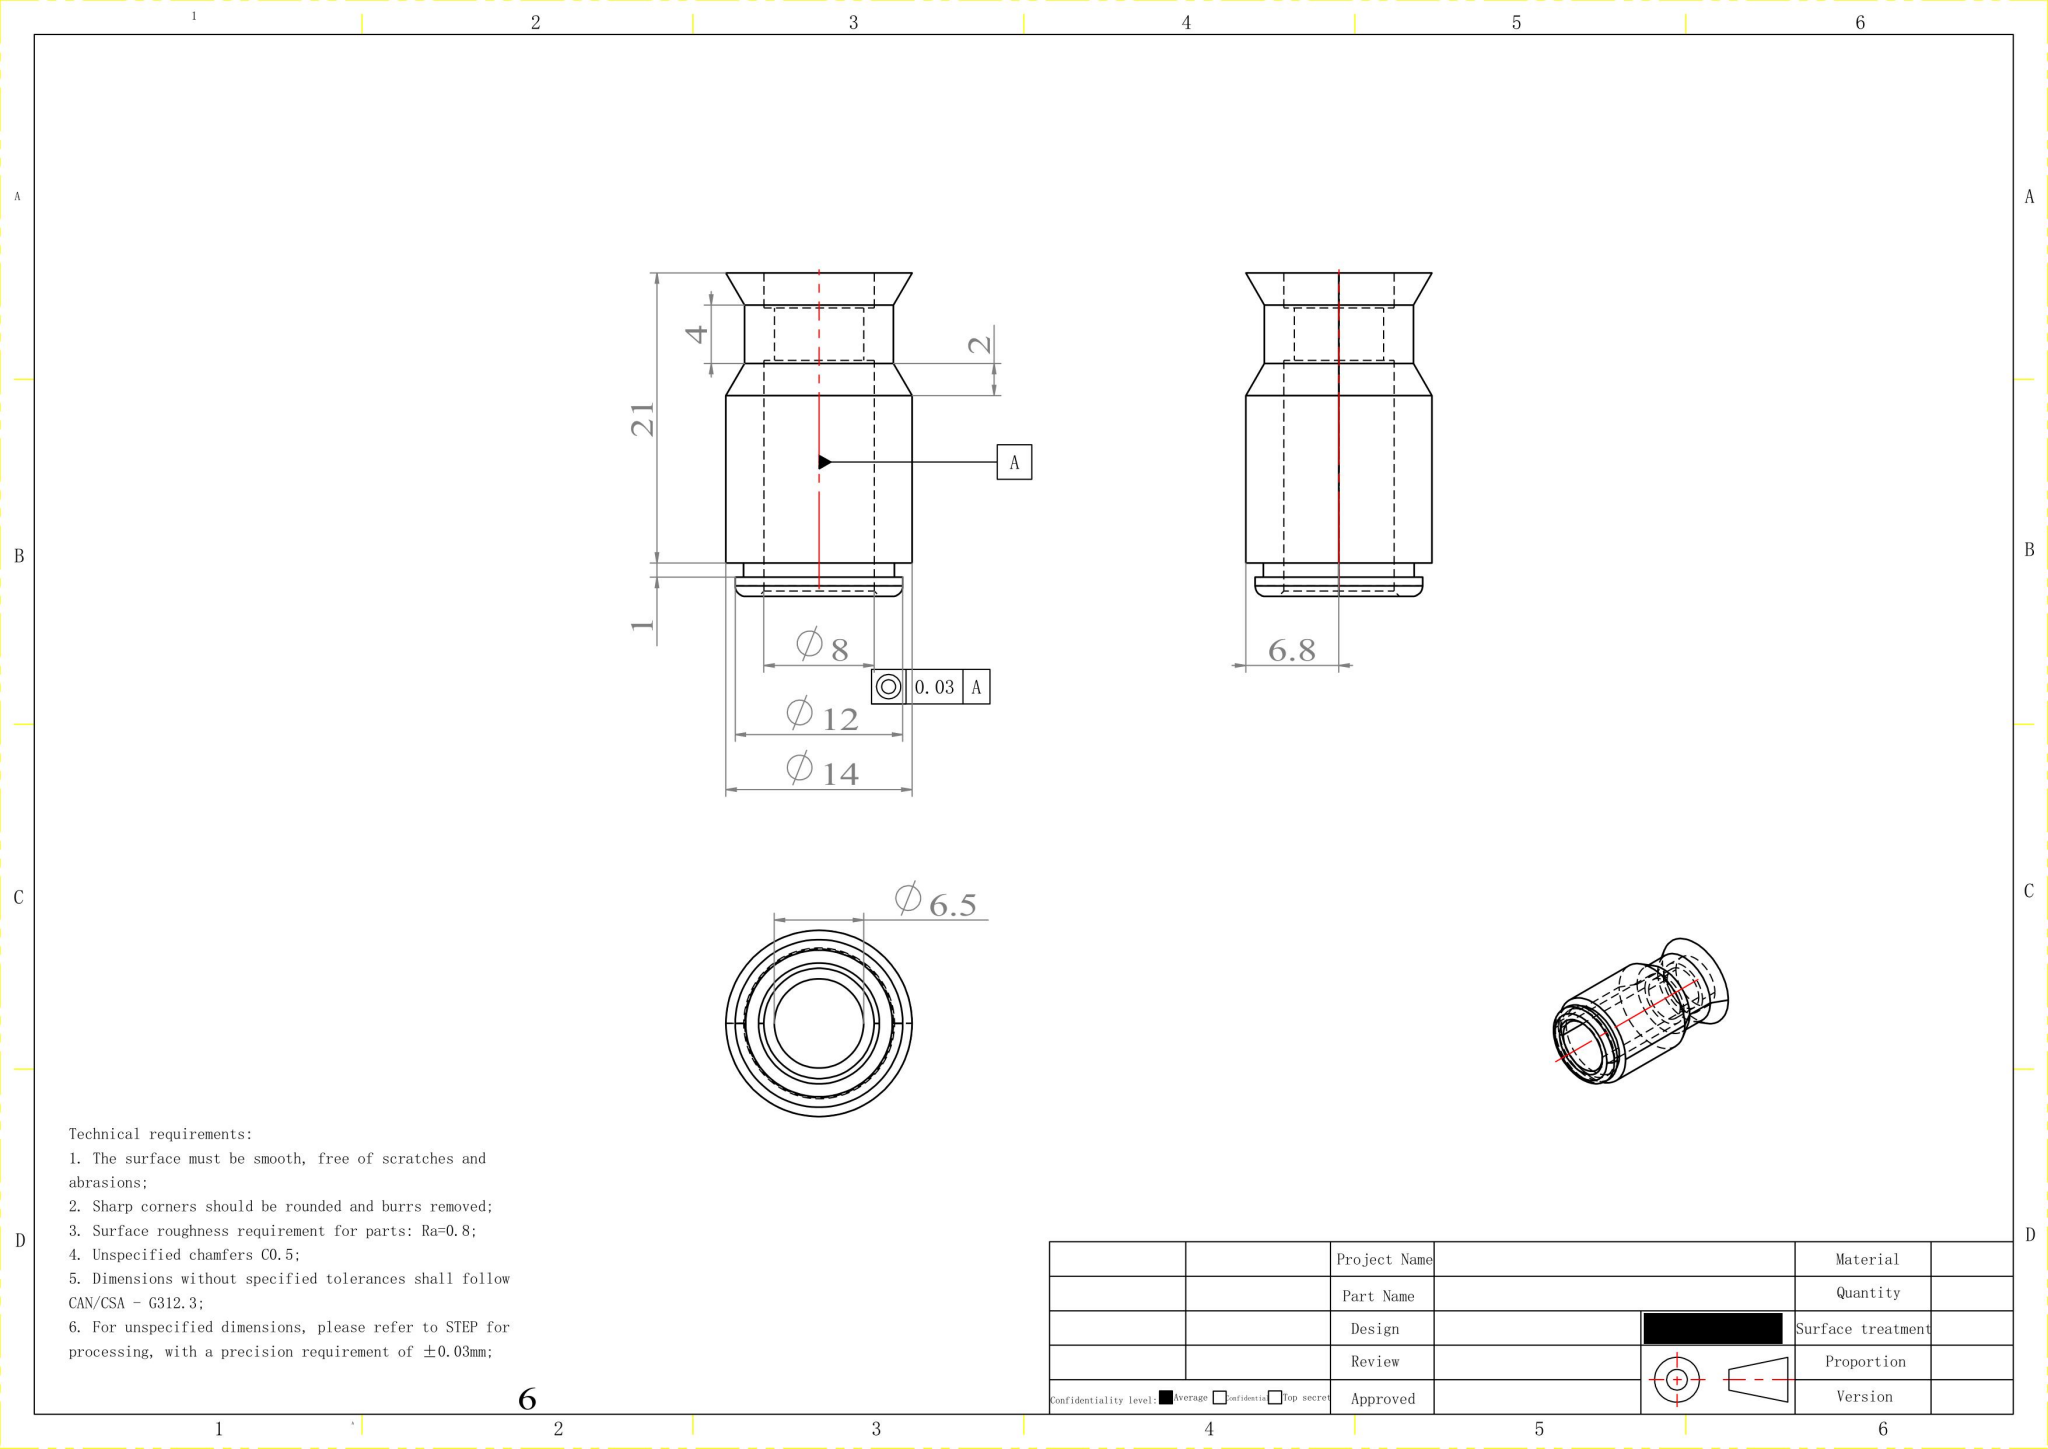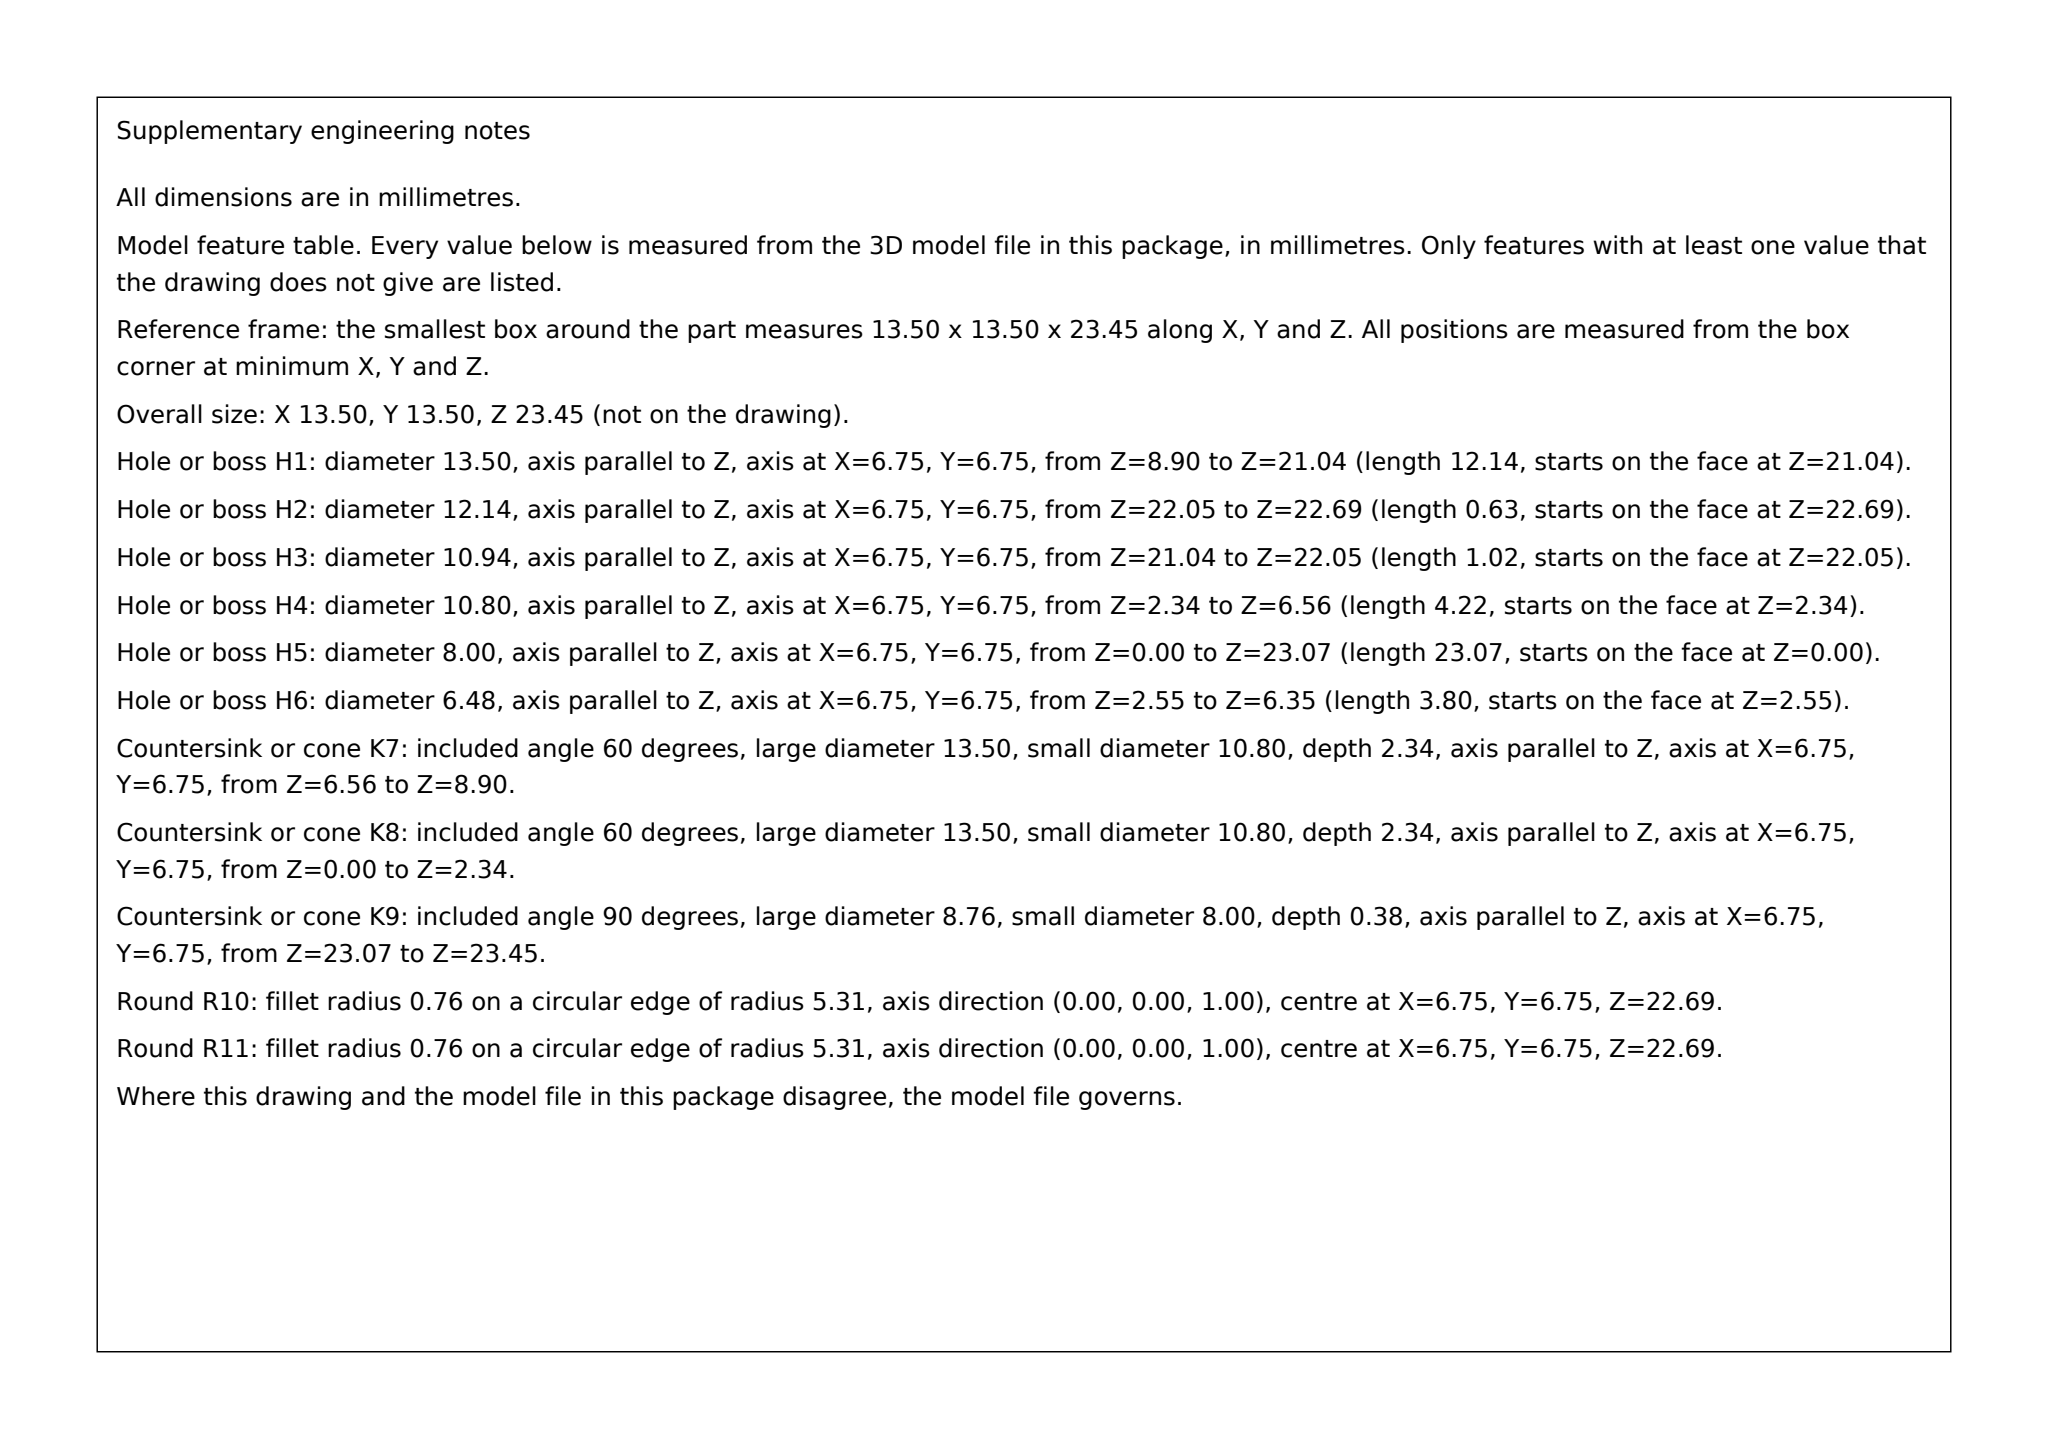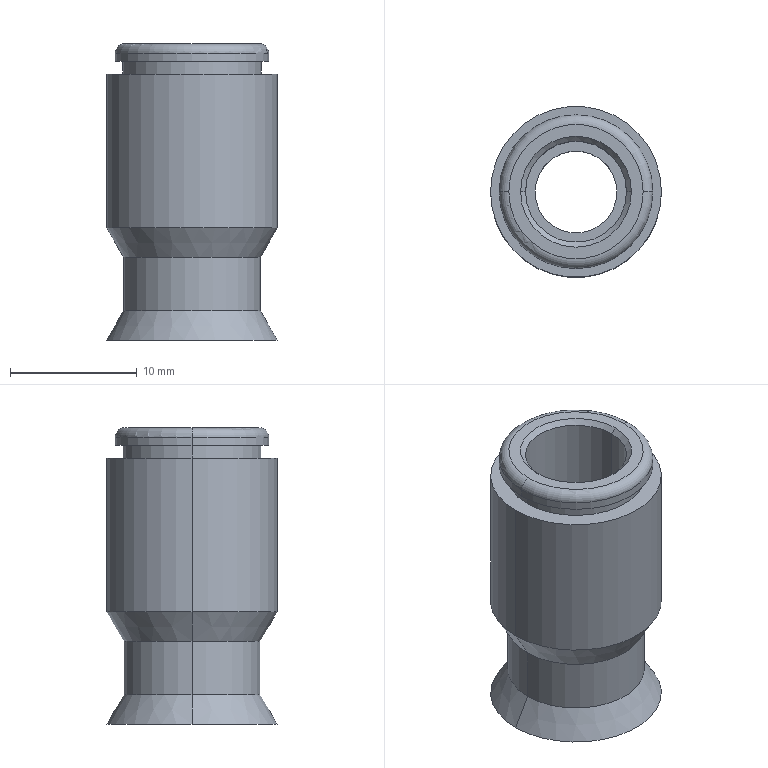Part | SolidWorks | mm | 1 solid | 28 faces | box 13.5 x 13.5 x 23.45 mm | volume 1807 mm3 | cylinder 14 | plane 6 | cone 6 | torus 2 | commonest cylinder face diameters 8 x4 6.476 x2 10.8 x2 13.5 x2 10.935 x2 12.15 x2
STEP:
#1=CARTESIAN_POINT('',(3.238,0.,1.9));
#2=VERTEX_POINT('',#1);
#3=CARTESIAN_POINT('',(-3.238,-0.,1.9));
#4=VERTEX_POINT('',#3);
#5=CARTESIAN_POINT('',(-0.,-0.,1.9));
#6=DIRECTION('',(0.,-0.,1.));
#7=DIRECTION('',(1.,0.,-0.));
#8=AXIS2_PLACEMENT_3D('',#5,#6,#7);
#9=CIRCLE('',#8,3.238);
#10=EDGE_CURVE('',#2,#4,#9,.T.);
#11=ORIENTED_EDGE('',*,*,#10,.F.);
#12=CARTESIAN_POINT('',(0.,0.,1.9));
#13=DIRECTION('',(-0.,0.,1.));
#14=DIRECTION('',(-1.,-0.,-0.));
#15=AXIS2_PLACEMENT_3D('',#12,#13,#14);
#16=CIRCLE('',#15,3.238);
#17=EDGE_CURVE('',#4,#2,#16,.T.);
#18=ORIENTED_EDGE('',*,*,#17,.F.);
#19=EDGE_LOOP('',(#11,#18));
#20=FACE_BOUND('',#19,.T.);
#21=CARTESIAN_POINT('',(4.,-0.,1.9));
#22=VERTEX_POINT('',#21);
#23=CARTESIAN_POINT('',(-4.,0.,1.9));
#24=VERTEX_POINT('',#23);
#25=CARTESIAN_POINT('',(0.,0.,1.9));
#26=DIRECTION('',(-0.,-0.,-1.));
#27=DIRECTION('',(1.,-0.,-0.));
#28=AXIS2_PLACEMENT_3D('',#25,#26,#27);
#29=CIRCLE('',#28,4.);
#30=EDGE_CURVE('',#22,#24,#29,.T.);
#31=ORIENTED_EDGE('',*,*,#30,.F.);
#32=CARTESIAN_POINT('',(0.,0.,1.9));
#33=DIRECTION('',(0.,0.,-1.));
#34=DIRECTION('',(-1.,0.,-0.));
#35=AXIS2_PLACEMENT_3D('',#32,#33,#34);
#36=CIRCLE('',#35,4.);
#37=EDGE_CURVE('',#24,#22,#36,.T.);
#38=ORIENTED_EDGE('',*,*,#37,.F.);
#39=EDGE_LOOP('',(#31,#38));
#40=FACE_OUTER_BOUND('',#39,.T.);
#41=CARTESIAN_POINT('',(0.,4.,1.9));
#42=DIRECTION('',(0.,0.,1.));
#43=DIRECTION('',(1.,0.,0.));
#44=AXIS2_PLACEMENT_3D('',#41,#42,#43);
#45=PLANE('',#44);
#46=ADVANCED_FACE('',(#20,#40),#45,.T.);
#47=CARTESIAN_POINT('',(-4.381,-0.,19.));
#48=VERTEX_POINT('',#47);
#49=CARTESIAN_POINT('',(4.381,0.,19.));
#50=VERTEX_POINT('',#49);
#51=CARTESIAN_POINT('',(0.,0.,19.));
#52=DIRECTION('',(0.,-0.,1.));
#53=DIRECTION('',(-1.,-0.,0.));
#54=AXIS2_PLACEMENT_3D('',#51,#52,#53);
#55=CIRCLE('',#54,4.381);
#56=EDGE_CURVE('',#48,#50,#55,.T.);
#57=ORIENTED_EDGE('',*,*,#56,.F.);
#58=CARTESIAN_POINT('',(0.,0.,19.));
#59=DIRECTION('',(0.,0.,1.));
#60=DIRECTION('',(1.,-0.,0.));
#61=AXIS2_PLACEMENT_3D('',#58,#59,#60);
#62=CIRCLE('',#61,4.381);
#63=EDGE_CURVE('',#50,#48,#62,.T.);
#64=ORIENTED_EDGE('',*,*,#63,.F.);
#65=EDGE_LOOP('',(#57,#64));
#66=FACE_BOUND('',#65,.T.);
#67=CARTESIAN_POINT('',(5.313,0.,19.));
#68=VERTEX_POINT('',#67);
#69=CARTESIAN_POINT('',(-5.313,0.,19.));
#70=VERTEX_POINT('',#69);
#71=CARTESIAN_POINT('',(0.,-0.,19.));
#72=DIRECTION('',(-0.,-0.,-1.));
#73=DIRECTION('',(1.,0.,-0.));
#74=AXIS2_PLACEMENT_3D('',#71,#72,#73);
#75=CIRCLE('',#74,5.313);
#76=EDGE_CURVE('',#68,#70,#75,.T.);
#77=ORIENTED_EDGE('',*,*,#76,.F.);
#78=CARTESIAN_POINT('',(0.,-0.,19.));
#79=DIRECTION('',(-0.,-0.,-1.));
#80=DIRECTION('',(-1.,0.,0.));
#81=AXIS2_PLACEMENT_3D('',#78,#79,#80);
#82=CIRCLE('',#81,5.313);
#83=EDGE_CURVE('',#70,#68,#82,.T.);
#84=ORIENTED_EDGE('',*,*,#83,.F.);
#85=EDGE_LOOP('',(#77,#84));
#86=FACE_OUTER_BOUND('',#85,.T.);
#87=CARTESIAN_POINT('',(0.,5.313,19.));
#88=DIRECTION('',(0.,0.,1.));
#89=DIRECTION('',(1.,0.,0.));
#90=AXIS2_PLACEMENT_3D('',#87,#88,#89);
#91=PLANE('',#90);
#92=ADVANCED_FACE('',(#66,#86),#91,.T.);
#93=CARTESIAN_POINT('',(5.468,0.,17.603));
#94=VERTEX_POINT('',#93);
#95=CARTESIAN_POINT('',(-5.468,0.,17.603));
#96=VERTEX_POINT('',#95);
#97=CARTESIAN_POINT('',(0.,-0.,17.603));
#98=DIRECTION('',(0.,0.,-1.));
#99=DIRECTION('',(1.,-0.,0.));
#100=AXIS2_PLACEMENT_3D('',#97,#98,#99);
#101=CIRCLE('',#100,5.468);
#102=EDGE_CURVE('',#94,#96,#101,.T.);
#103=ORIENTED_EDGE('',*,*,#102,.F.);
#104=CARTESIAN_POINT('',(0.,-0.,17.603));
#105=DIRECTION('',(-0.,-0.,-1.));
#106=DIRECTION('',(-1.,0.,0.));
#107=AXIS2_PLACEMENT_3D('',#104,#105,#106);
#108=CIRCLE('',#107,5.468);
#109=EDGE_CURVE('',#96,#94,#108,.T.);
#110=ORIENTED_EDGE('',*,*,#109,.F.);
#111=EDGE_LOOP('',(#103,#110));
#112=FACE_BOUND('',#111,.T.);
#113=CARTESIAN_POINT('',(6.075,-0.,17.603));
#114=VERTEX_POINT('',#113);
#115=CARTESIAN_POINT('',(-6.075,0.,17.603));
#116=VERTEX_POINT('',#115);
#117=CARTESIAN_POINT('',(0.,0.,17.603));
#118=DIRECTION('',(-0.,-0.,1.));
#119=DIRECTION('',(1.,-0.,0.));
#120=AXIS2_PLACEMENT_3D('',#117,#118,#119);
#121=CIRCLE('',#120,6.075);
#122=EDGE_CURVE('',#114,#116,#121,.T.);
#123=ORIENTED_EDGE('',*,*,#122,.F.);
#124=CARTESIAN_POINT('',(0.,0.,17.603));
#125=DIRECTION('',(-0.,-0.,1.));
#126=DIRECTION('',(-1.,0.,0.));
#127=AXIS2_PLACEMENT_3D('',#124,#125,#126);
#128=CIRCLE('',#127,6.075);
#129=EDGE_CURVE('',#116,#114,#128,.T.);
#130=ORIENTED_EDGE('',*,*,#129,.F.);
#131=EDGE_LOOP('',(#123,#130));
#132=FACE_OUTER_BOUND('',#131,.T.);
#133=CARTESIAN_POINT('',(0.,6.075,17.603));
#134=DIRECTION('',(0.,0.,-1.));
#135=DIRECTION('',(0.,-1.,0.));
#136=AXIS2_PLACEMENT_3D('',#133,#134,#135);
#137=PLANE('',#136);
#138=ADVANCED_FACE('',(#112,#132),#137,.T.);
#139=CARTESIAN_POINT('',(5.468,-0.,16.587));
#140=VERTEX_POINT('',#139);
#141=CARTESIAN_POINT('',(-5.468,0.,16.587));
#142=VERTEX_POINT('',#141);
#143=CARTESIAN_POINT('',(0.,-0.,16.587));
#144=DIRECTION('',(0.,0.,1.));
#145=DIRECTION('',(1.,-0.,0.));
#146=AXIS2_PLACEMENT_3D('',#143,#144,#145);
#147=CIRCLE('',#146,5.468);
#148=EDGE_CURVE('',#140,#142,#147,.T.);
#149=ORIENTED_EDGE('',*,*,#148,.F.);
#150=CARTESIAN_POINT('',(-0.,-0.,16.587));
#151=DIRECTION('',(0.,0.,1.));
#152=DIRECTION('',(-1.,0.,0.));
#153=AXIS2_PLACEMENT_3D('',#150,#151,#152);
#154=CIRCLE('',#153,5.468);
#155=EDGE_CURVE('',#142,#140,#154,.T.);
#156=ORIENTED_EDGE('',*,*,#155,.F.);
#157=EDGE_LOOP('',(#149,#156));
#158=FACE_BOUND('',#157,.T.);
#159=CARTESIAN_POINT('',(6.75,0.,16.587));
#160=VERTEX_POINT('',#159);
#161=CARTESIAN_POINT('',(-6.75,0.,16.587));
#162=VERTEX_POINT('',#161);
#163=CARTESIAN_POINT('',(0.,0.,16.587));
#164=DIRECTION('',(0.,0.,-1.));
#165=DIRECTION('',(1.,-0.,0.));
#166=AXIS2_PLACEMENT_3D('',#163,#164,#165);
#167=CIRCLE('',#166,6.75);
#168=EDGE_CURVE('',#160,#162,#167,.T.);
#169=ORIENTED_EDGE('',*,*,#168,.F.);
#170=CARTESIAN_POINT('',(0.,0.,16.587));
#171=DIRECTION('',(0.,0.,-1.));
#172=DIRECTION('',(-1.,0.,0.));
#173=AXIS2_PLACEMENT_3D('',#170,#171,#172);
#174=CIRCLE('',#173,6.75);
#175=EDGE_CURVE('',#162,#160,#174,.T.);
#176=ORIENTED_EDGE('',*,*,#175,.F.);
#177=EDGE_LOOP('',(#169,#176));
#178=FACE_OUTER_BOUND('',#177,.T.);
#179=CARTESIAN_POINT('',(0.,6.75,16.587));
#180=DIRECTION('',(0.,0.,1.));
#181=DIRECTION('',(1.,0.,0.));
#182=AXIS2_PLACEMENT_3D('',#179,#180,#181);
#183=PLANE('',#182);
#184=ADVANCED_FACE('',(#158,#178),#183,.T.);
#185=CARTESIAN_POINT('',(3.238,0.,-1.9));
#186=VERTEX_POINT('',#185);
#187=CARTESIAN_POINT('',(-3.238,-0.,-1.9));
#188=VERTEX_POINT('',#187);
#189=CARTESIAN_POINT('',(-0.,-0.,-1.9));
#190=DIRECTION('',(0.,-0.,-1.));
#191=DIRECTION('',(1.,0.,0.));
#192=AXIS2_PLACEMENT_3D('',#189,#190,#191);
#193=CIRCLE('',#192,3.238);
#194=EDGE_CURVE('',#186,#188,#193,.T.);
#195=ORIENTED_EDGE('',*,*,#194,.F.);
#196=CARTESIAN_POINT('',(0.,0.,-1.9));
#197=DIRECTION('',(-0.,-0.,-1.));
#198=DIRECTION('',(-1.,-0.,0.));
#199=AXIS2_PLACEMENT_3D('',#196,#197,#198);
#200=CIRCLE('',#199,3.238);
#201=EDGE_CURVE('',#188,#186,#200,.T.);
#202=ORIENTED_EDGE('',*,*,#201,.F.);
#203=EDGE_LOOP('',(#195,#202));
#204=FACE_BOUND('',#203,.T.);
#205=CARTESIAN_POINT('',(4.,-0.,-1.9));
#206=VERTEX_POINT('',#205);
#207=CARTESIAN_POINT('',(-4.,-0.,-1.9));
#208=VERTEX_POINT('',#207);
#209=CARTESIAN_POINT('',(0.,-0.,-1.9));
#210=DIRECTION('',(-0.,-0.,1.));
#211=DIRECTION('',(1.,0.,0.));
#212=AXIS2_PLACEMENT_3D('',#209,#210,#211);
#213=CIRCLE('',#212,4.);
#214=EDGE_CURVE('',#206,#208,#213,.T.);
#215=ORIENTED_EDGE('',*,*,#214,.F.);
#216=CARTESIAN_POINT('',(-0.,-0.,-1.9));
#217=DIRECTION('',(0.,-0.,1.));
#218=DIRECTION('',(-1.,0.,0.));
#219=AXIS2_PLACEMENT_3D('',#216,#217,#218);
#220=CIRCLE('',#219,4.);
#221=EDGE_CURVE('',#208,#206,#220,.T.);
#222=ORIENTED_EDGE('',*,*,#221,.F.);
#223=EDGE_LOOP('',(#215,#222));
#224=FACE_OUTER_BOUND('',#223,.T.);
#225=CARTESIAN_POINT('',(0.,4.,-1.9));
#226=DIRECTION('',(0.,0.,-1.));
#227=DIRECTION('',(0.,-1.,0.));
#228=AXIS2_PLACEMENT_3D('',#225,#226,#227);
#229=PLANE('',#228);
#230=ADVANCED_FACE('',(#204,#224),#229,.T.);
#231=CARTESIAN_POINT('',(-6.75,-0.,-4.449));
#232=VERTEX_POINT('',#231);
#233=CARTESIAN_POINT('',(6.75,0.,-4.449));
#234=VERTEX_POINT('',#233);
#235=CARTESIAN_POINT('',(0.,0.,-4.449));
#236=DIRECTION('',(0.,0.,-1.));
#237=DIRECTION('',(-1.,-0.,0.));
#238=AXIS2_PLACEMENT_3D('',#235,#236,#237);
#239=CIRCLE('',#238,6.75);
#240=EDGE_CURVE('',#232,#234,#239,.T.);
#241=ORIENTED_EDGE('',*,*,#240,.F.);
#242=CARTESIAN_POINT('',(-5.4,-0.,-2.111));
#243=VERTEX_POINT('',#242);
#244=CARTESIAN_POINT('',(-5.4,0.,-2.111));
#245=DIRECTION('',(-0.5,0.,-0.866));
#246=VECTOR('',#245,1000.);
#247=LINE('',#244,#246);
#248=EDGE_CURVE('',#243,#232,#247,.T.);
#249=ORIENTED_EDGE('',*,*,#248,.F.);
#250=CARTESIAN_POINT('',(5.4,0.,-2.111));
#251=VERTEX_POINT('',#250);
#252=CARTESIAN_POINT('',(0.,0.,-2.111));
#253=DIRECTION('',(-0.,0.,1.));
#254=DIRECTION('',(1.,0.,0.));
#255=AXIS2_PLACEMENT_3D('',#252,#253,#254);
#256=CIRCLE('',#255,5.4);
#257=EDGE_CURVE('',#251,#243,#256,.T.);
#258=ORIENTED_EDGE('',*,*,#257,.F.);
#259=CARTESIAN_POINT('',(6.75,0.,-4.449));
#260=DIRECTION('',(-0.5,-0.,0.866));
#261=VECTOR('',#260,1000.);
#262=LINE('',#259,#261);
#263=EDGE_CURVE('',#234,#251,#262,.T.);
#264=ORIENTED_EDGE('',*,*,#263,.F.);
#265=EDGE_LOOP('',(#241,#249,#258,#264));
#266=FACE_OUTER_BOUND('',#265,.T.);
#267=CARTESIAN_POINT('',(0.,0.,6.242));
#268=DIRECTION('',(0.,0.,-1.));
#269=DIRECTION('',(-1.,-0.,0.));
#270=AXIS2_PLACEMENT_3D('',#267,#268,#269);
#271=CONICAL_SURFACE('',#270,0.5774,0.5236);
#272=ADVANCED_FACE('',(#266),#271,.T.);
#273=ORIENTED_EDGE('',*,*,#263,.T.);
#274=CARTESIAN_POINT('',(-0.,-0.,-2.111));
#275=DIRECTION('',(0.,-0.,1.));
#276=DIRECTION('',(-1.,-0.,0.));
#277=AXIS2_PLACEMENT_3D('',#274,#275,#276);
#278=CIRCLE('',#277,5.4);
#279=EDGE_CURVE('',#243,#251,#278,.T.);
#280=ORIENTED_EDGE('',*,*,#279,.F.);
#281=ORIENTED_EDGE('',*,*,#248,.T.);
#282=CARTESIAN_POINT('',(-0.,0.,-4.449));
#283=DIRECTION('',(0.,0.,-1.));
#284=DIRECTION('',(1.,-0.,0.));
#285=AXIS2_PLACEMENT_3D('',#282,#283,#284);
#286=CIRCLE('',#285,6.75);
#287=EDGE_CURVE('',#234,#232,#286,.T.);
#288=ORIENTED_EDGE('',*,*,#287,.F.);
#289=EDGE_LOOP('',(#273,#280,#281,#288));
#290=FACE_OUTER_BOUND('',#289,.T.);
#291=CARTESIAN_POINT('',(0.,0.,6.242));
#292=DIRECTION('',(0.,0.,-1.));
#293=DIRECTION('',(-1.,-0.,0.));
#294=AXIS2_PLACEMENT_3D('',#291,#292,#293);
#295=CONICAL_SURFACE('',#294,0.5774,0.5236);
#296=ADVANCED_FACE('',(#290),#295,.T.);
#297=CARTESIAN_POINT('',(4.,0.,-4.449));
#298=VERTEX_POINT('',#297);
#299=CARTESIAN_POINT('',(-4.,0.,-4.449));
#300=VERTEX_POINT('',#299);
#301=CARTESIAN_POINT('',(0.,-0.,-4.449));
#302=DIRECTION('',(0.,0.,1.));
#303=DIRECTION('',(1.,-0.,0.));
#304=AXIS2_PLACEMENT_3D('',#301,#302,#303);
#305=CIRCLE('',#304,4.);
#306=EDGE_CURVE('',#298,#300,#305,.T.);
#307=ORIENTED_EDGE('',*,*,#306,.F.);
#308=CARTESIAN_POINT('',(4.,0.,-1.9));
#309=DIRECTION('',(0.,0.,-1.));
#310=VECTOR('',#309,1000.);
#311=LINE('',#308,#310);
#312=EDGE_CURVE('',#206,#298,#311,.T.);
#313=ORIENTED_EDGE('',*,*,#312,.F.);
#314=ORIENTED_EDGE('',*,*,#214,.T.);
#315=CARTESIAN_POINT('',(-4.,0.,-4.449));
#316=DIRECTION('',(0.,-0.,1.));
#317=VECTOR('',#316,1000.);
#318=LINE('',#315,#317);
#319=EDGE_CURVE('',#300,#208,#318,.T.);
#320=ORIENTED_EDGE('',*,*,#319,.F.);
#321=EDGE_LOOP('',(#307,#313,#314,#320));
#322=FACE_OUTER_BOUND('',#321,.T.);
#323=CARTESIAN_POINT('',(0.,-0.,-4.449));
#324=DIRECTION('',(-0.,0.,1.));
#325=DIRECTION('',(1.,0.,0.));
#326=AXIS2_PLACEMENT_3D('',#323,#324,#325);
#327=CYLINDRICAL_SURFACE('',#326,4.);
#328=ADVANCED_FACE('',(#322),#327,.F.);
#329=ORIENTED_EDGE('',*,*,#319,.T.);
#330=ORIENTED_EDGE('',*,*,#221,.T.);
#331=ORIENTED_EDGE('',*,*,#312,.T.);
#332=CARTESIAN_POINT('',(-0.,-0.,-4.449));
#333=DIRECTION('',(0.,0.,1.));
#334=DIRECTION('',(-1.,0.,0.));
#335=AXIS2_PLACEMENT_3D('',#332,#333,#334);
#336=CIRCLE('',#335,4.);
#337=EDGE_CURVE('',#300,#298,#336,.T.);
#338=ORIENTED_EDGE('',*,*,#337,.F.);
#339=EDGE_LOOP('',(#329,#330,#331,#338));
#340=FACE_OUTER_BOUND('',#339,.T.);
#341=CARTESIAN_POINT('',(0.,-0.,-4.449));
#342=DIRECTION('',(-0.,0.,1.));
#343=DIRECTION('',(1.,0.,0.));
#344=AXIS2_PLACEMENT_3D('',#341,#342,#343);
#345=CYLINDRICAL_SURFACE('',#344,4.);
#346=ADVANCED_FACE('',(#340),#345,.F.);
#347=ORIENTED_EDGE('',*,*,#201,.T.);
#348=CARTESIAN_POINT('',(3.238,0.,1.9));
#349=DIRECTION('',(0.,0.,-1.));
#350=VECTOR('',#349,1000.);
#351=LINE('',#348,#350);
#352=EDGE_CURVE('',#2,#186,#351,.T.);
#353=ORIENTED_EDGE('',*,*,#352,.F.);
#354=ORIENTED_EDGE('',*,*,#10,.T.);
#355=CARTESIAN_POINT('',(-3.238,-0.,-1.9));
#356=DIRECTION('',(0.,0.,1.));
#357=VECTOR('',#356,1000.);
#358=LINE('',#355,#357);
#359=EDGE_CURVE('',#188,#4,#358,.T.);
#360=ORIENTED_EDGE('',*,*,#359,.F.);
#361=EDGE_LOOP('',(#347,#353,#354,#360));
#362=FACE_OUTER_BOUND('',#361,.T.);
#363=CARTESIAN_POINT('',(0.,0.,-1.9));
#364=DIRECTION('',(-0.,0.,1.));
#365=DIRECTION('',(1.,-0.,0.));
#366=AXIS2_PLACEMENT_3D('',#363,#364,#365);
#367=CYLINDRICAL_SURFACE('',#366,3.238);
#368=ADVANCED_FACE('',(#362),#367,.F.);
#369=ORIENTED_EDGE('',*,*,#359,.T.);
#370=ORIENTED_EDGE('',*,*,#17,.T.);
#371=ORIENTED_EDGE('',*,*,#352,.T.);
#372=ORIENTED_EDGE('',*,*,#194,.T.);
#373=EDGE_LOOP('',(#369,#370,#371,#372));
#374=FACE_OUTER_BOUND('',#373,.T.);
#375=CARTESIAN_POINT('',(0.,0.,-1.9));
#376=DIRECTION('',(-0.,0.,1.));
#377=DIRECTION('',(1.,-0.,0.));
#378=AXIS2_PLACEMENT_3D('',#375,#376,#377);
#379=CYLINDRICAL_SURFACE('',#378,3.238);
#380=ADVANCED_FACE('',(#374),#379,.F.);
#381=CARTESIAN_POINT('',(-5.4,0.,2.111));
#382=VERTEX_POINT('',#381);
#383=CARTESIAN_POINT('',(5.4,0.,2.111));
#384=VERTEX_POINT('',#383);
#385=CARTESIAN_POINT('',(-0.,-0.,2.111));
#386=DIRECTION('',(0.,0.,1.));
#387=DIRECTION('',(-1.,0.,0.));
#388=AXIS2_PLACEMENT_3D('',#385,#386,#387);
#389=CIRCLE('',#388,5.4);
#390=EDGE_CURVE('',#382,#384,#389,.T.);
#391=ORIENTED_EDGE('',*,*,#390,.F.);
#392=CARTESIAN_POINT('',(-5.4,0.,2.111));
#393=DIRECTION('',(0.,-0.,-1.));
#394=VECTOR('',#393,1000.);
#395=LINE('',#392,#394);
#396=EDGE_CURVE('',#382,#243,#395,.T.);
#397=ORIENTED_EDGE('',*,*,#396,.T.);
#398=ORIENTED_EDGE('',*,*,#279,.T.);
#399=CARTESIAN_POINT('',(5.4,0.,2.111));
#400=DIRECTION('',(0.,0.,-1.));
#401=VECTOR('',#400,1000.);
#402=LINE('',#399,#401);
#403=EDGE_CURVE('',#384,#251,#402,.T.);
#404=ORIENTED_EDGE('',*,*,#403,.F.);
#405=EDGE_LOOP('',(#391,#397,#398,#404));
#406=FACE_OUTER_BOUND('',#405,.T.);
#407=CARTESIAN_POINT('',(0.,-0.,-2.111));
#408=DIRECTION('',(-0.,-0.,1.));
#409=DIRECTION('',(1.,0.,0.));
#410=AXIS2_PLACEMENT_3D('',#407,#408,#409);
#411=CYLINDRICAL_SURFACE('',#410,5.4);
#412=ADVANCED_FACE('',(#406),#411,.T.);
#413=ORIENTED_EDGE('',*,*,#257,.T.);
#414=ORIENTED_EDGE('',*,*,#396,.F.);
#415=CARTESIAN_POINT('',(0.,0.,2.111));
#416=DIRECTION('',(0.,-0.,1.));
#417=DIRECTION('',(1.,0.,0.));
#418=AXIS2_PLACEMENT_3D('',#415,#416,#417);
#419=CIRCLE('',#418,5.4);
#420=EDGE_CURVE('',#384,#382,#419,.T.);
#421=ORIENTED_EDGE('',*,*,#420,.F.);
#422=ORIENTED_EDGE('',*,*,#403,.T.);
#423=EDGE_LOOP('',(#413,#414,#421,#422));
#424=FACE_OUTER_BOUND('',#423,.T.);
#425=CARTESIAN_POINT('',(0.,-0.,-2.111));
#426=DIRECTION('',(-0.,-0.,1.));
#427=DIRECTION('',(1.,0.,0.));
#428=AXIS2_PLACEMENT_3D('',#425,#426,#427);
#429=CYLINDRICAL_SURFACE('',#428,5.4);
#430=ADVANCED_FACE('',(#424),#429,.T.);
#431=CARTESIAN_POINT('',(6.75,-0.,4.449));
#432=VERTEX_POINT('',#431);
#433=CARTESIAN_POINT('',(-6.75,0.,4.449));
#434=VERTEX_POINT('',#433);
#435=CARTESIAN_POINT('',(0.,-0.,4.449));
#436=DIRECTION('',(0.,0.,1.));
#437=DIRECTION('',(1.,0.,0.));
#438=AXIS2_PLACEMENT_3D('',#435,#436,#437);
#439=CIRCLE('',#438,6.75);
#440=EDGE_CURVE('',#432,#434,#439,.T.);
#441=ORIENTED_EDGE('',*,*,#440,.F.);
#442=CARTESIAN_POINT('',(6.75,-0.,4.449));
#443=DIRECTION('',(-0.5,0.,-0.866));
#444=VECTOR('',#443,1000.);
#445=LINE('',#442,#444);
#446=EDGE_CURVE('',#432,#384,#445,.T.);
#447=ORIENTED_EDGE('',*,*,#446,.T.);
#448=ORIENTED_EDGE('',*,*,#420,.T.);
#449=CARTESIAN_POINT('',(-6.75,0.,4.449));
#450=DIRECTION('',(0.5,0.,-0.866));
#451=VECTOR('',#450,1000.);
#452=LINE('',#449,#451);
#453=EDGE_CURVE('',#434,#382,#452,.T.);
#454=ORIENTED_EDGE('',*,*,#453,.F.);
#455=EDGE_LOOP('',(#441,#447,#448,#454));
#456=FACE_OUTER_BOUND('',#455,.T.);
#457=CARTESIAN_POINT('',(0.,-0.,-6.242));
#458=DIRECTION('',(0.,-0.,1.));
#459=DIRECTION('',(-1.,0.,0.));
#460=AXIS2_PLACEMENT_3D('',#457,#458,#459);
#461=CONICAL_SURFACE('',#460,0.5774,0.5236);
#462=ADVANCED_FACE('',(#456),#461,.T.);
#463=ORIENTED_EDGE('',*,*,#390,.T.);
#464=ORIENTED_EDGE('',*,*,#446,.F.);
#465=CARTESIAN_POINT('',(0.,0.,4.449));
#466=DIRECTION('',(0.,0.,1.));
#467=DIRECTION('',(-1.,-0.,0.));
#468=AXIS2_PLACEMENT_3D('',#465,#466,#467);
#469=CIRCLE('',#468,6.75);
#470=EDGE_CURVE('',#434,#432,#469,.T.);
#471=ORIENTED_EDGE('',*,*,#470,.F.);
#472=ORIENTED_EDGE('',*,*,#453,.T.);
#473=EDGE_LOOP('',(#463,#464,#471,#472));
#474=FACE_OUTER_BOUND('',#473,.T.);
#475=CARTESIAN_POINT('',(0.,-0.,-6.242));
#476=DIRECTION('',(0.,-0.,1.));
#477=DIRECTION('',(-1.,0.,0.));
#478=AXIS2_PLACEMENT_3D('',#475,#476,#477);
#479=CONICAL_SURFACE('',#478,0.5774,0.5236);
#480=ADVANCED_FACE('',(#474),#479,.T.);
#481=ORIENTED_EDGE('',*,*,#440,.T.);
#482=CARTESIAN_POINT('',(-6.75,0.,4.449));
#483=DIRECTION('',(0.,0.,1.));
#484=VECTOR('',#483,1000.);
#485=LINE('',#482,#484);
#486=EDGE_CURVE('',#434,#162,#485,.T.);
#487=ORIENTED_EDGE('',*,*,#486,.T.);
#488=ORIENTED_EDGE('',*,*,#175,.T.);
#489=CARTESIAN_POINT('',(6.75,0.,4.449));
#490=DIRECTION('',(-0.,0.,1.));
#491=VECTOR('',#490,1000.);
#492=LINE('',#489,#491);
#493=EDGE_CURVE('',#432,#160,#492,.T.);
#494=ORIENTED_EDGE('',*,*,#493,.F.);
#495=EDGE_LOOP('',(#481,#487,#488,#494));
#496=FACE_OUTER_BOUND('',#495,.T.);
#497=CARTESIAN_POINT('',(-0.,0.,16.587));
#498=DIRECTION('',(0.,0.,-1.));
#499=DIRECTION('',(1.,0.,0.));
#500=AXIS2_PLACEMENT_3D('',#497,#498,#499);
#501=CYLINDRICAL_SURFACE('',#500,6.75);
#502=ADVANCED_FACE('',(#496),#501,.T.);
#503=ORIENTED_EDGE('',*,*,#486,.F.);
#504=ORIENTED_EDGE('',*,*,#470,.T.);
#505=ORIENTED_EDGE('',*,*,#493,.T.);
#506=ORIENTED_EDGE('',*,*,#168,.T.);
#507=EDGE_LOOP('',(#503,#504,#505,#506));
#508=FACE_OUTER_BOUND('',#507,.T.);
#509=CARTESIAN_POINT('',(-0.,0.,16.587));
#510=DIRECTION('',(0.,0.,-1.));
#511=DIRECTION('',(1.,0.,0.));
#512=AXIS2_PLACEMENT_3D('',#509,#510,#511);
#513=CYLINDRICAL_SURFACE('',#512,6.75);
#514=ADVANCED_FACE('',(#508),#513,.T.);
#515=ORIENTED_EDGE('',*,*,#155,.T.);
#516=CARTESIAN_POINT('',(5.468,0.,17.603));
#517=DIRECTION('',(0.,0.,-1.));
#518=VECTOR('',#517,1000.);
#519=LINE('',#516,#518);
#520=EDGE_CURVE('',#94,#140,#519,.T.);
#521=ORIENTED_EDGE('',*,*,#520,.F.);
#522=ORIENTED_EDGE('',*,*,#102,.T.);
#523=CARTESIAN_POINT('',(-5.468,0.,16.587));
#524=DIRECTION('',(0.,0.,1.));
#525=VECTOR('',#524,1000.);
#526=LINE('',#523,#525);
#527=EDGE_CURVE('',#142,#96,#526,.T.);
#528=ORIENTED_EDGE('',*,*,#527,.F.);
#529=EDGE_LOOP('',(#515,#521,#522,#528));
#530=FACE_OUTER_BOUND('',#529,.T.);
#531=CARTESIAN_POINT('',(-0.,0.,17.603));
#532=DIRECTION('',(0.,0.,-1.));
#533=DIRECTION('',(1.,0.,0.));
#534=AXIS2_PLACEMENT_3D('',#531,#532,#533);
#535=CYLINDRICAL_SURFACE('',#534,5.468);
#536=ADVANCED_FACE('',(#530),#535,.T.);
#537=ORIENTED_EDGE('',*,*,#527,.T.);
#538=ORIENTED_EDGE('',*,*,#109,.T.);
#539=ORIENTED_EDGE('',*,*,#520,.T.);
#540=ORIENTED_EDGE('',*,*,#148,.T.);
#541=EDGE_LOOP('',(#537,#538,#539,#540));
#542=FACE_OUTER_BOUND('',#541,.T.);
#543=CARTESIAN_POINT('',(-0.,0.,17.603));
#544=DIRECTION('',(0.,0.,-1.));
#545=DIRECTION('',(1.,0.,0.));
#546=AXIS2_PLACEMENT_3D('',#543,#544,#545);
#547=CYLINDRICAL_SURFACE('',#546,5.468);
#548=ADVANCED_FACE('',(#542),#547,.T.);
#549=ORIENTED_EDGE('',*,*,#129,.T.);
#550=CARTESIAN_POINT('',(6.075,-0.,18.238));
#551=VERTEX_POINT('',#550);
#552=CARTESIAN_POINT('',(6.075,0.,18.238));
#553=DIRECTION('',(0.,0.,-1.));
#554=VECTOR('',#553,1000.);
#555=LINE('',#552,#554);
#556=EDGE_CURVE('',#551,#114,#555,.T.);
#557=ORIENTED_EDGE('',*,*,#556,.F.);
#558=CARTESIAN_POINT('',(-6.075,0.,18.238));
#559=VERTEX_POINT('',#558);
#560=CARTESIAN_POINT('',(0.,0.,18.238));
#561=DIRECTION('',(-0.,-0.,1.));
#562=DIRECTION('',(-1.,0.,0.));
#563=AXIS2_PLACEMENT_3D('',#560,#561,#562);
#564=CIRCLE('',#563,6.075);
#565=EDGE_CURVE('',#559,#551,#564,.T.);
#566=ORIENTED_EDGE('',*,*,#565,.F.);
#567=CARTESIAN_POINT('',(-6.075,0.,17.603));
#568=DIRECTION('',(0.,0.,1.));
#569=VECTOR('',#568,1000.);
#570=LINE('',#567,#569);
#571=EDGE_CURVE('',#116,#559,#570,.T.);
#572=ORIENTED_EDGE('',*,*,#571,.F.);
#573=EDGE_LOOP('',(#549,#557,#566,#572));
#574=FACE_OUTER_BOUND('',#573,.T.);
#575=CARTESIAN_POINT('',(-0.,-0.,18.238));
#576=DIRECTION('',(0.,0.,-1.));
#577=DIRECTION('',(1.,0.,0.));
#578=AXIS2_PLACEMENT_3D('',#575,#576,#577);
#579=CYLINDRICAL_SURFACE('',#578,6.075);
#580=ADVANCED_FACE('',(#574),#579,.T.);
#581=ORIENTED_EDGE('',*,*,#571,.T.);
#582=CARTESIAN_POINT('',(-0.,0.,18.238));
#583=DIRECTION('',(-0.,-0.,-1.));
#584=DIRECTION('',(-1.,0.,0.));
#585=AXIS2_PLACEMENT_3D('',#582,#583,#584);
#586=CIRCLE('',#585,6.075);
#587=EDGE_CURVE('',#559,#551,#586,.T.);
#588=ORIENTED_EDGE('',*,*,#587,.T.);
#589=ORIENTED_EDGE('',*,*,#556,.T.);
#590=ORIENTED_EDGE('',*,*,#122,.T.);
#591=EDGE_LOOP('',(#581,#588,#589,#590));
#592=FACE_OUTER_BOUND('',#591,.T.);
#593=CARTESIAN_POINT('',(-0.,-0.,18.238));
#594=DIRECTION('',(0.,0.,-1.));
#595=DIRECTION('',(1.,0.,0.));
#596=AXIS2_PLACEMENT_3D('',#593,#594,#595);
#597=CYLINDRICAL_SURFACE('',#596,6.075);
#598=ADVANCED_FACE('',(#592),#597,.T.);
#599=ORIENTED_EDGE('',*,*,#565,.T.);
#600=CARTESIAN_POINT('',(5.313,0.,18.238));
#601=DIRECTION('',(0.,1.,0.));
#602=DIRECTION('',(0.00004509,0.,1.));
#603=AXIS2_PLACEMENT_3D('',#600,#601,#602);
#604=CIRCLE('',#603,0.762);
#605=EDGE_CURVE('',#68,#551,#604,.T.);
#606=ORIENTED_EDGE('',*,*,#605,.F.);
#607=ORIENTED_EDGE('',*,*,#76,.T.);
#608=CARTESIAN_POINT('',(-5.313,0.,18.238));
#609=DIRECTION('',(0.,1.,0.));
#610=DIRECTION('',(-1.,0.,0.));
#611=AXIS2_PLACEMENT_3D('',#608,#609,#610);
#612=CIRCLE('',#611,0.762);
#613=EDGE_CURVE('',#559,#70,#612,.T.);
#614=ORIENTED_EDGE('',*,*,#613,.F.);
#615=EDGE_LOOP('',(#599,#606,#607,#614));
#616=FACE_OUTER_BOUND('',#615,.T.);
#617=CARTESIAN_POINT('',(-0.,0.,18.238));
#618=DIRECTION('',(0.,0.,1.));
#619=DIRECTION('',(1.,-0.,-0.));
#620=AXIS2_PLACEMENT_3D('',#617,#618,#619);
#621=TOROIDAL_SURFACE('',#620,5.313,0.762);
#622=ADVANCED_FACE('',(#616),#621,.T.);
#623=ORIENTED_EDGE('',*,*,#613,.T.);
#624=ORIENTED_EDGE('',*,*,#83,.T.);
#625=ORIENTED_EDGE('',*,*,#605,.T.);
#626=ORIENTED_EDGE('',*,*,#587,.F.);
#627=EDGE_LOOP('',(#623,#624,#625,#626));
#628=FACE_OUTER_BOUND('',#627,.T.);
#629=CARTESIAN_POINT('',(-0.,0.,18.238));
#630=DIRECTION('',(0.,0.,1.));
#631=DIRECTION('',(1.,-0.,-0.));
#632=AXIS2_PLACEMENT_3D('',#629,#630,#631);
#633=TOROIDAL_SURFACE('',#632,5.313,0.762);
#634=ADVANCED_FACE('',(#628),#633,.T.);
#635=CARTESIAN_POINT('',(4.,-0.,18.619));
#636=VERTEX_POINT('',#635);
#637=CARTESIAN_POINT('',(-4.,0.,18.619));
#638=VERTEX_POINT('',#637);
#639=CARTESIAN_POINT('',(-0.,0.,18.619));
#640=DIRECTION('',(0.,0.,1.));
#641=DIRECTION('',(1.,-0.,0.));
#642=AXIS2_PLACEMENT_3D('',#639,#640,#641);
#643=CIRCLE('',#642,4.);
#644=EDGE_CURVE('',#636,#638,#643,.T.);
#645=ORIENTED_EDGE('',*,*,#644,.F.);
#646=CARTESIAN_POINT('',(4.,-0.,18.619));
#647=DIRECTION('',(0.7071,0.,0.7071));
#648=VECTOR('',#647,1000.);
#649=LINE('',#646,#648);
#650=EDGE_CURVE('',#636,#50,#649,.T.);
#651=ORIENTED_EDGE('',*,*,#650,.T.);
#652=ORIENTED_EDGE('',*,*,#63,.T.);
#653=CARTESIAN_POINT('',(-4.,0.,18.619));
#654=DIRECTION('',(-0.7071,0.,0.7071));
#655=VECTOR('',#654,1000.);
#656=LINE('',#653,#655);
#657=EDGE_CURVE('',#638,#48,#656,.T.);
#658=ORIENTED_EDGE('',*,*,#657,.F.);
#659=EDGE_LOOP('',(#645,#651,#652,#658));
#660=FACE_OUTER_BOUND('',#659,.T.);
#661=CARTESIAN_POINT('',(0.,0.,15.619));
#662=DIRECTION('',(0.,0.,1.));
#663=DIRECTION('',(-1.,0.,0.));
#664=AXIS2_PLACEMENT_3D('',#661,#662,#663);
#665=CONICAL_SURFACE('',#664,1.,0.7854);
#666=ADVANCED_FACE('',(#660),#665,.F.);
#667=ORIENTED_EDGE('',*,*,#650,.F.);
#668=CARTESIAN_POINT('',(0.,0.,18.619));
#669=DIRECTION('',(-0.,-0.,1.));
#670=DIRECTION('',(-1.,0.,0.));
#671=AXIS2_PLACEMENT_3D('',#668,#669,#670);
#672=CIRCLE('',#671,4.);
#673=EDGE_CURVE('',#638,#636,#672,.T.);
#674=ORIENTED_EDGE('',*,*,#673,.F.);
#675=ORIENTED_EDGE('',*,*,#657,.T.);
#676=ORIENTED_EDGE('',*,*,#56,.T.);
#677=EDGE_LOOP('',(#667,#674,#675,#676));
#678=FACE_OUTER_BOUND('',#677,.T.);
#679=CARTESIAN_POINT('',(0.,0.,15.619));
#680=DIRECTION('',(0.,0.,1.));
#681=DIRECTION('',(-1.,0.,0.));
#682=AXIS2_PLACEMENT_3D('',#679,#680,#681);
#683=CONICAL_SURFACE('',#682,1.,0.7854);
#684=ADVANCED_FACE('',(#678),#683,.F.);
#685=ORIENTED_EDGE('',*,*,#644,.T.);
#686=CARTESIAN_POINT('',(-4.,0.,18.619));
#687=DIRECTION('',(0.,0.,-1.));
#688=VECTOR('',#687,1000.);
#689=LINE('',#686,#688);
#690=EDGE_CURVE('',#638,#24,#689,.T.);
#691=ORIENTED_EDGE('',*,*,#690,.T.);
#692=ORIENTED_EDGE('',*,*,#37,.T.);
#693=CARTESIAN_POINT('',(4.,0.,18.619));
#694=DIRECTION('',(0.,0.,-1.));
#695=VECTOR('',#694,1000.);
#696=LINE('',#693,#695);
#697=EDGE_CURVE('',#636,#22,#696,.T.);
#698=ORIENTED_EDGE('',*,*,#697,.F.);
#699=EDGE_LOOP('',(#685,#691,#692,#698));
#700=FACE_OUTER_BOUND('',#699,.T.);
#701=CARTESIAN_POINT('',(-0.,0.,18.619));
#702=DIRECTION('',(0.,0.,-1.));
#703=DIRECTION('',(1.,0.,0.));
#704=AXIS2_PLACEMENT_3D('',#701,#702,#703);
#705=CYLINDRICAL_SURFACE('',#704,4.);
#706=ADVANCED_FACE('',(#700),#705,.F.);
#707=ORIENTED_EDGE('',*,*,#690,.F.);
#708=ORIENTED_EDGE('',*,*,#673,.T.);
#709=ORIENTED_EDGE('',*,*,#697,.T.);
#710=ORIENTED_EDGE('',*,*,#30,.T.);
#711=EDGE_LOOP('',(#707,#708,#709,#710));
#712=FACE_OUTER_BOUND('',#711,.T.);
#713=CARTESIAN_POINT('',(-0.,0.,18.619));
#714=DIRECTION('',(0.,0.,-1.));
#715=DIRECTION('',(1.,0.,0.));
#716=AXIS2_PLACEMENT_3D('',#713,#714,#715);
#717=CYLINDRICAL_SURFACE('',#716,4.);
#718=ADVANCED_FACE('',(#712),#717,.F.);
#719=ORIENTED_EDGE('',*,*,#337,.T.);
#720=ORIENTED_EDGE('',*,*,#306,.T.);
#721=EDGE_LOOP('',(#719,#720));
#722=FACE_BOUND('',#721,.T.);
#723=ORIENTED_EDGE('',*,*,#287,.T.);
#724=ORIENTED_EDGE('',*,*,#240,.T.);
#725=EDGE_LOOP('',(#723,#724));
#726=FACE_OUTER_BOUND('',#725,.T.);
#727=CARTESIAN_POINT('',(0.,0.,-4.449));
#728=DIRECTION('',(0.,0.,-1.));
#729=DIRECTION('',(0.,-1.,0.));
#730=AXIS2_PLACEMENT_3D('',#727,#728,#729);
#731=PLANE('',#730);
#732=ADVANCED_FACE('',(#722,#726),#731,.T.);
#733=CLOSED_SHELL('',(#46,#92,#138,#184,#230,#272,#296,#328,#346,#368,#380,#412,#430,#462,#480,#502,#514,#536,#548,#580,#598,#622,#634,#666,#684,#706,#718,#732));
#734=MANIFOLD_SOLID_BREP('',#733);
#735=CARTESIAN_POINT('',(0.,0.,0.));
#736=DIRECTION('',(0.,0.,1.));
#737=DIRECTION('',(1.,0.,0.));
#738=AXIS2_PLACEMENT_3D('',#735,#736,#737);
#739=(LENGTH_UNIT()NAMED_UNIT(*)SI_UNIT(.MILLI.,.METRE.));
#740=UNCERTAINTY_MEASURE_WITH_UNIT(LENGTH_MEASURE(0.00001),#739,'','');
#741=(NAMED_UNIT(*)PLANE_ANGLE_UNIT()SI_UNIT($,.RADIAN.));
#742=(NAMED_UNIT(*)SI_UNIT($,.STERADIAN.)SOLID_ANGLE_UNIT());
#743=(GEOMETRIC_REPRESENTATION_CONTEXT(3)GLOBAL_UNCERTAINTY_ASSIGNED_CONTEXT((#740))GLOBAL_UNIT_ASSIGNED_CONTEXT((#739,#741,#742))REPRESENTATION_CONTEXT('',''));
#744=ADVANCED_BREP_SHAPE_REPRESENTATION('',(#734,#738),#743);